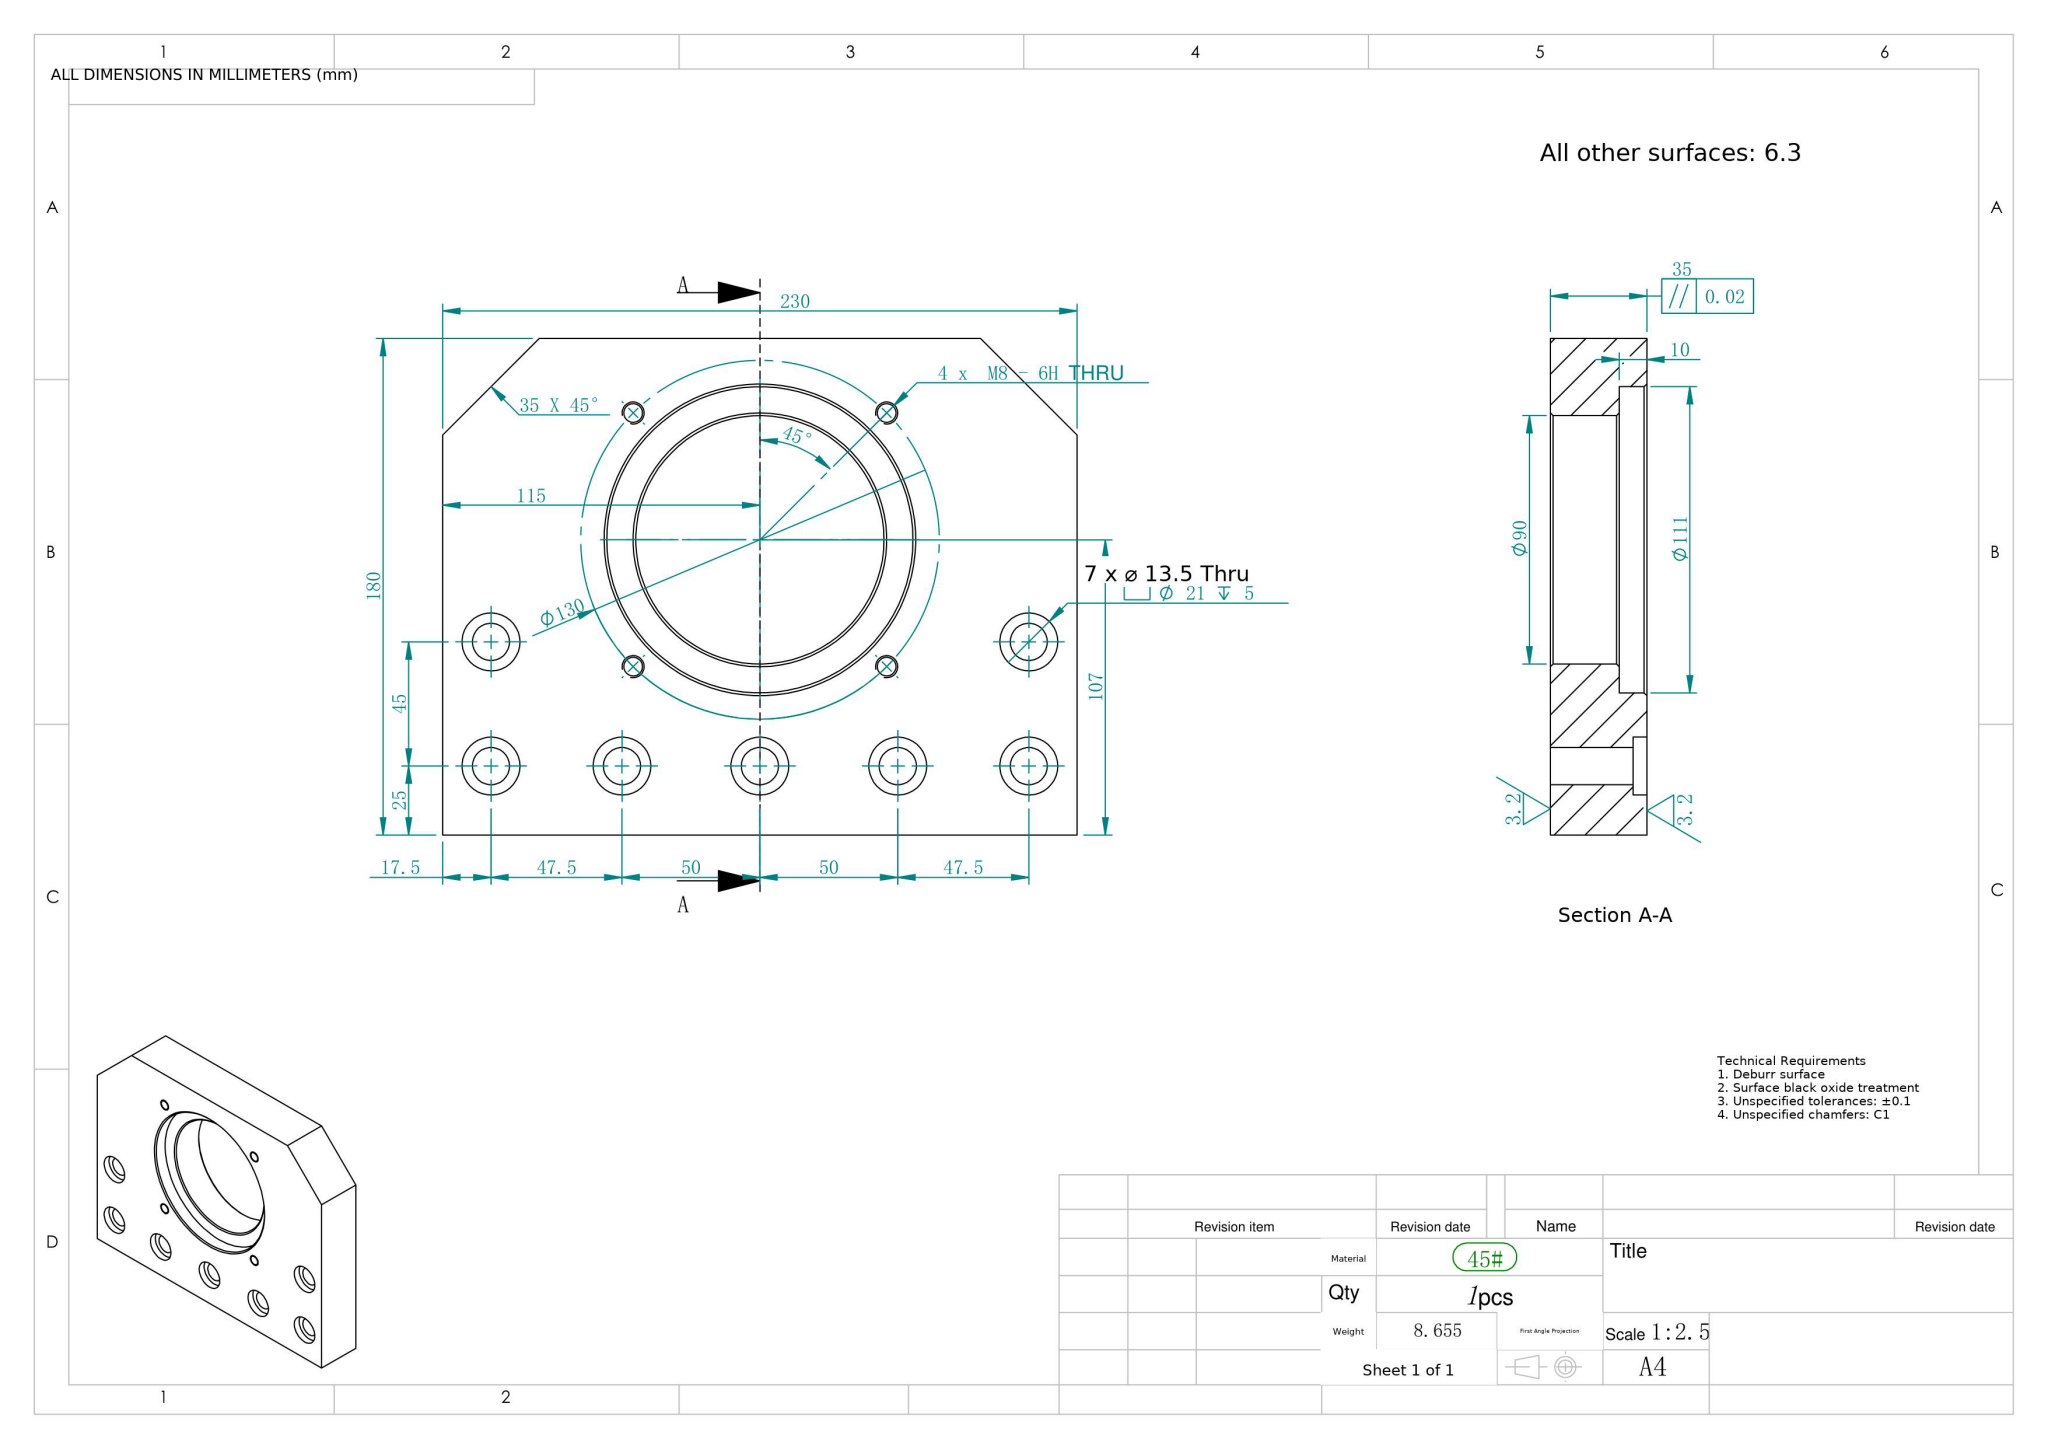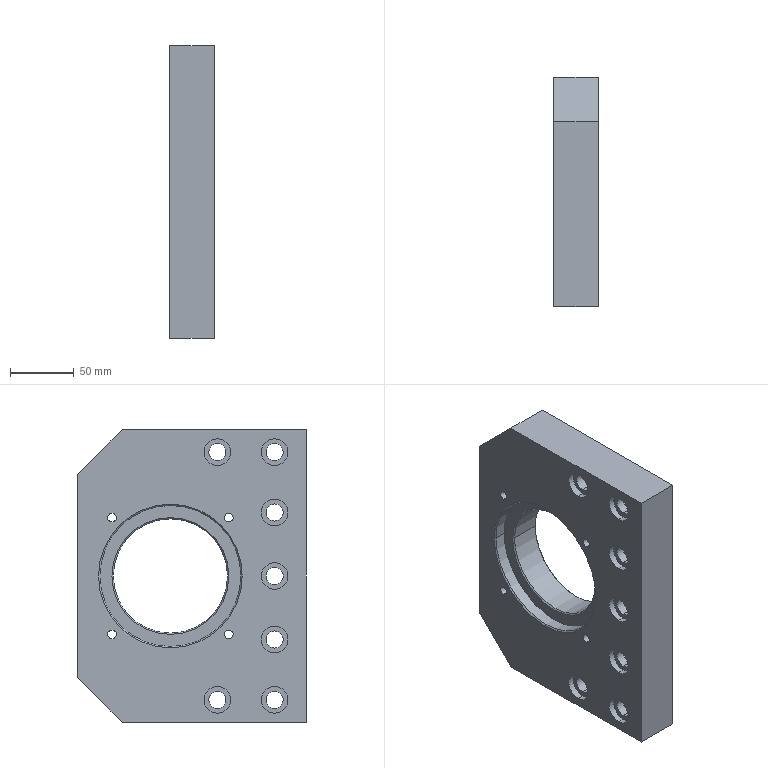Part | NX | mm | 1 solid | 62 faces | box 35 x 180 x 230 mm | volume 1102587 mm3 | cylinder 40 | plane 16 | cone 6 | commonest cylinder face diameters 21 x14 13.5 x14 6.8 x8 90 x2 111 x2